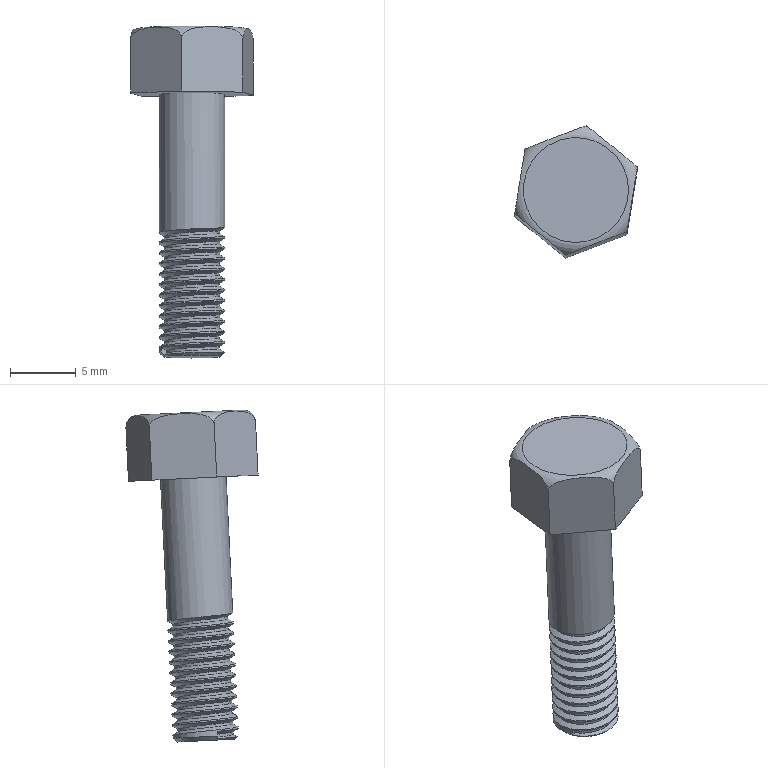Component | NX | CCJ-024_3 | 2 solids | 29 faces | volume 689 mm3 | cylinder 13 | plane 12 | spline 2 | cone 1 | torus 1 | commonest cylinder face diameters 5 x12 4.2 x1